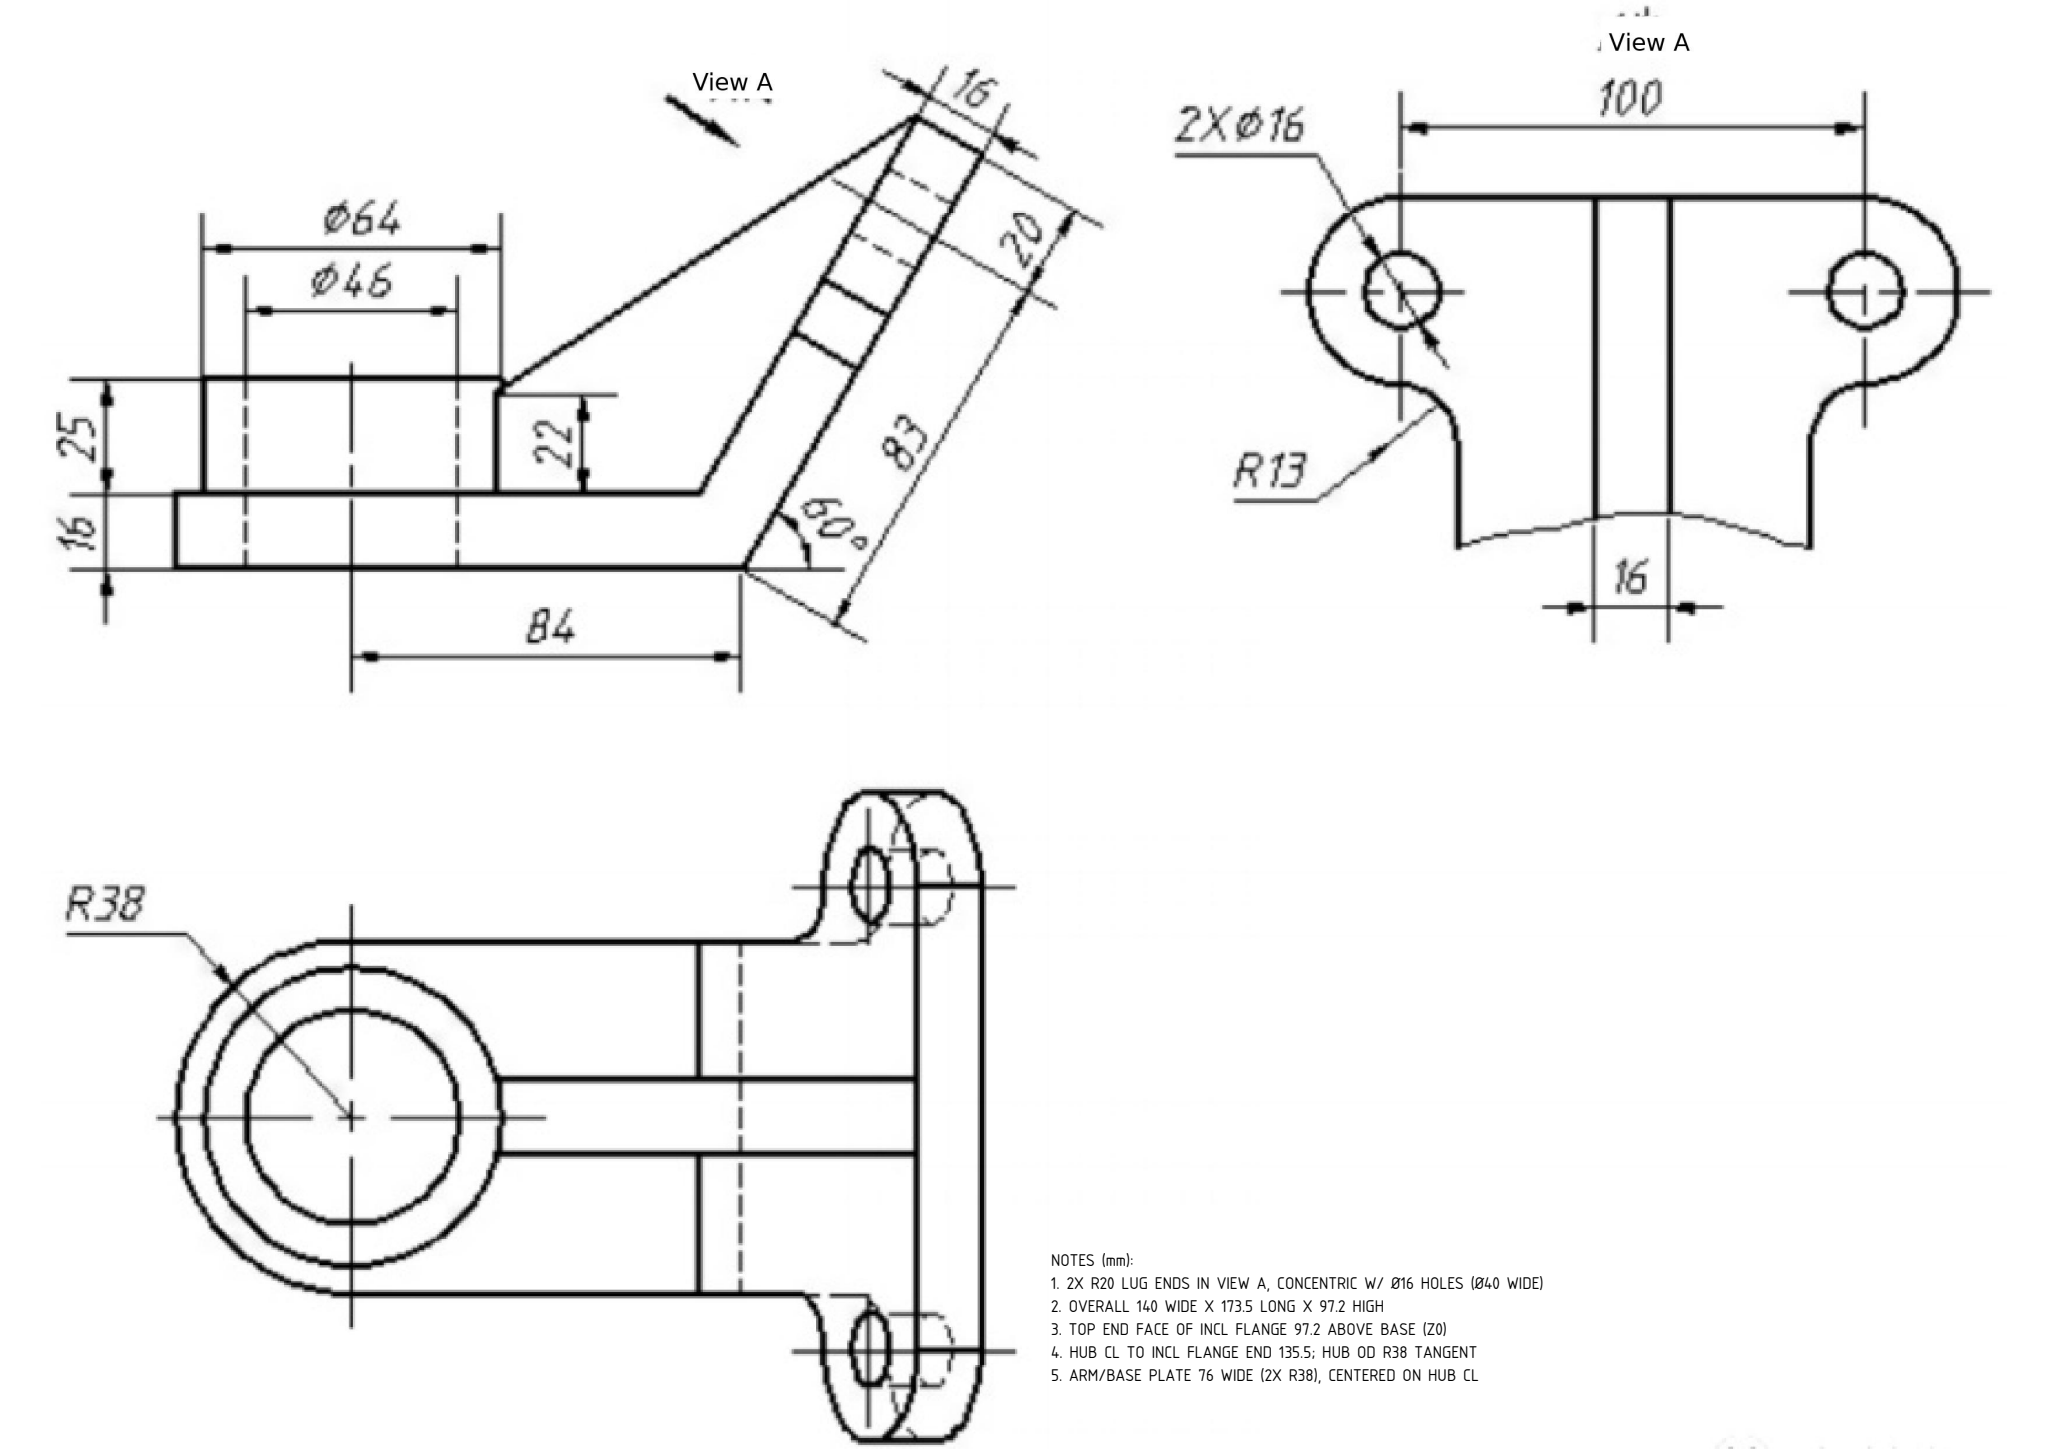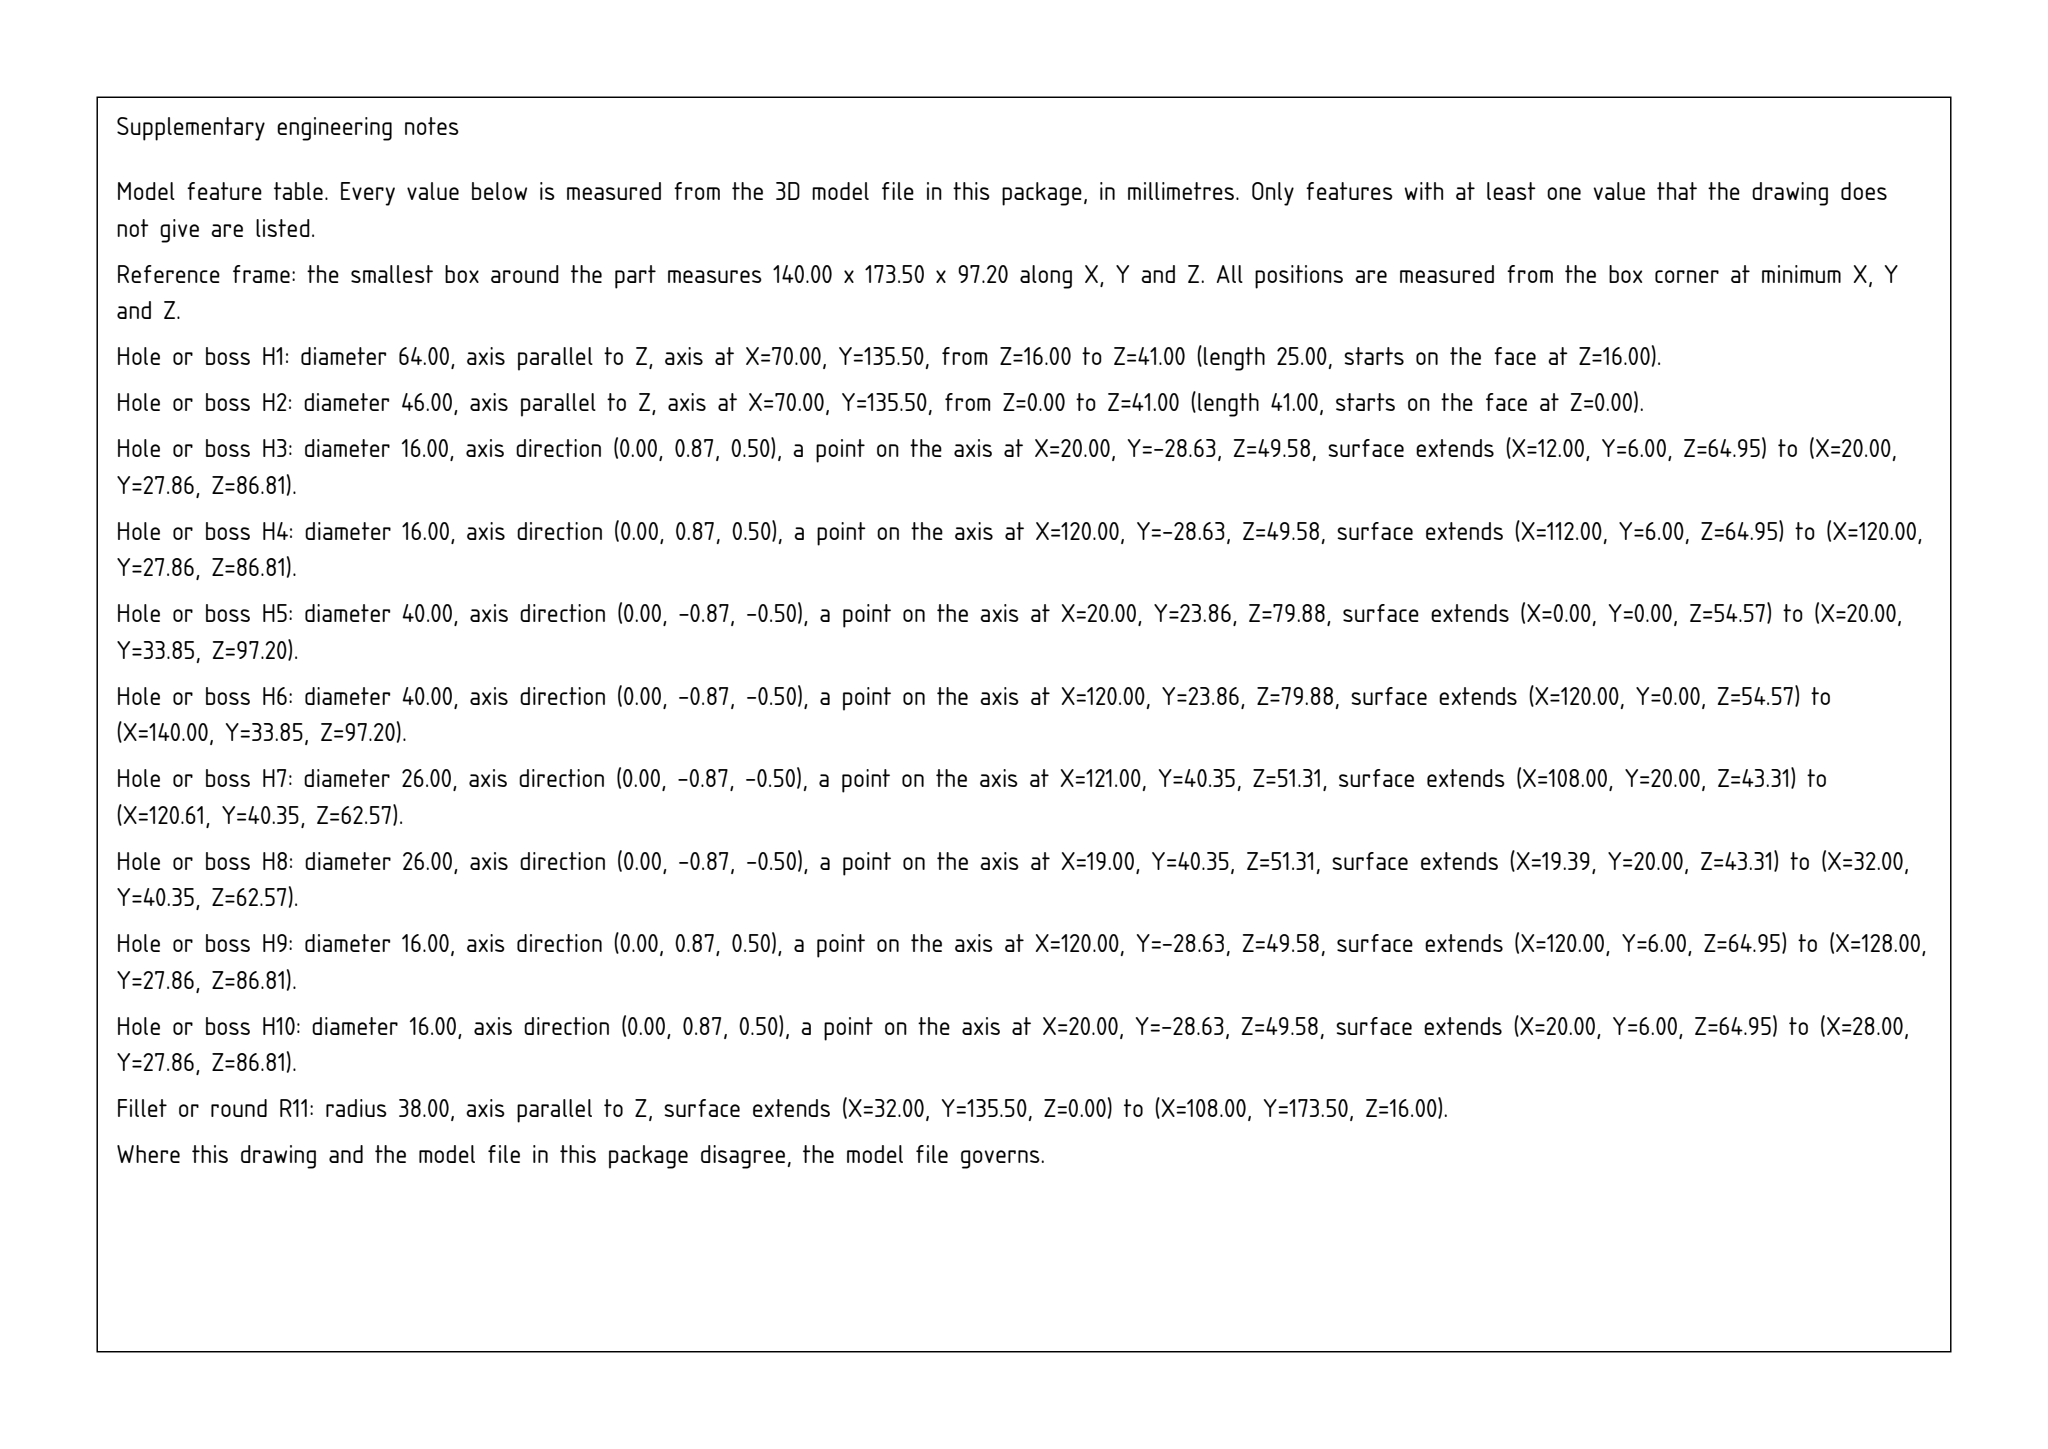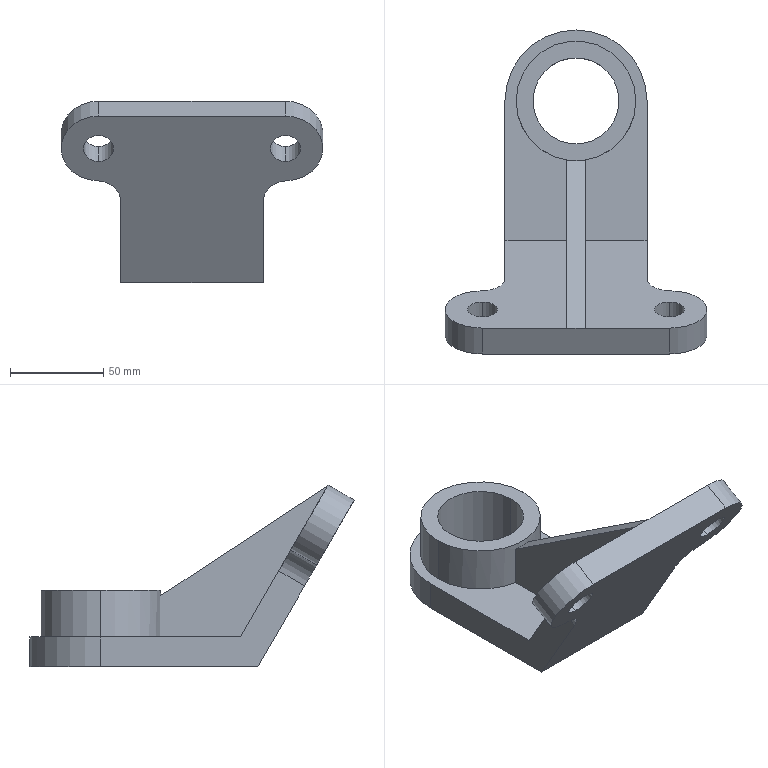Part | SolidWorks | mm | 1 solid | 25 faces | box 140 x 173.5 x 97.2 mm | volume 322175 mm3 | cylinder 13 | plane 12 | commonest cylinder face diameters 16 x4 46 x2 64 x2 40 x2 26 x2 76 x1
Drawing notes:
2X R20 LUG ENDS IN VIEW A, CONCENTRIC W/ Ø16 HOLES (Ø40 WIDE) | from the solid: Ø40 cyl, axis Y, at x=20 and x=120 (same x as the 2X Ø16 holes) -> R20 rounded lug ends, 100 apart
OVERALL 140 WIDE X 173.5 LONG X 97.2 HIGH | from the solid: bbox_xyz = [140.0, 173.5, 97.201]
TOP END FACE OF INCL FLANGE 97.2 ABOVE BASE (Z0) | from the solid: bbox Z max = 97.201 above base plane z=0; base bottom plane z=0.0
HUB CL TO INCL FLANGE END 135.5; HUB OD R38 TANGENT | from the solid: Ø46/Ø64/Ø76 hub axis at y=135.5 from bbox y-min; bbox y = 173.5 = 135.5 + 38
ARM/BASE PLATE 76 WIDE (2X R38), CENTERED ON HUB CL | from the solid: x-normal planes at 32.0 and 108.0 (76 apart) symmetric about hub axis x=70; Ø76 cyl, axis Z, pos (70,135.5), L=16
STEP:
#1=CARTESIAN_POINT('',(-50.,-121.5,64.952));
#2=VERTEX_POINT('',#1);
#3=CARTESIAN_POINT('',(-50.,-129.5,78.808));
#4=VERTEX_POINT('',#3);
#5=CARTESIAN_POINT('',(-50.,-125.5,71.88));
#6=DIRECTION('',(0.,0.866,0.5));
#7=DIRECTION('',(0.,-0.5,0.866));
#8=AXIS2_PLACEMENT_3D('',#5,#6,#7);
#9=CIRCLE('',#8,8.);
#10=EDGE_CURVE('',#2,#4,#9,.T.);
#11=ORIENTED_EDGE('',*,*,#10,.F.);
#12=CARTESIAN_POINT('',(-50.,-107.644,72.952));
#13=VERTEX_POINT('',#12);
#14=CARTESIAN_POINT('',(-50.,-160.125,42.652));
#15=DIRECTION('',(0.,0.866,0.5));
#16=VECTOR('',#15,1000.);
#17=LINE('',#14,#16);
#18=EDGE_CURVE('',#2,#13,#17,.T.);
#19=ORIENTED_EDGE('',*,*,#18,.T.);
#20=CARTESIAN_POINT('',(-50.,-115.644,86.808));
#21=VERTEX_POINT('',#20);
#22=CARTESIAN_POINT('',(-50.,-111.644,79.88));
#23=DIRECTION('',(0.,0.866,0.5));
#24=DIRECTION('',(0.,-0.5,0.866));
#25=AXIS2_PLACEMENT_3D('',#22,#23,#24);
#26=CIRCLE('',#25,8.);
#27=EDGE_CURVE('',#13,#21,#26,.T.);
#28=ORIENTED_EDGE('',*,*,#27,.T.);
#29=CARTESIAN_POINT('',(-50.,-168.125,56.508));
#30=DIRECTION('',(0.,0.866,0.5));
#31=VECTOR('',#30,1000.);
#32=LINE('',#29,#31);
#33=EDGE_CURVE('',#4,#21,#32,.T.);
#34=ORIENTED_EDGE('',*,*,#33,.F.);
#35=EDGE_LOOP('',(#11,#19,#28,#34));
#36=FACE_OUTER_BOUND('',#35,.T.);
#37=CARTESIAN_POINT('',(-50.,-164.125,49.58));
#38=DIRECTION('',(0.,0.866,0.5));
#39=DIRECTION('',(0.,-0.5,0.866));
#40=AXIS2_PLACEMENT_3D('',#37,#38,#39);
#41=CYLINDRICAL_SURFACE('',#40,8.);
#42=ADVANCED_FACE('',(#36),#41,.F.);
#43=CARTESIAN_POINT('',(50.,-121.5,64.952));
#44=VERTEX_POINT('',#43);
#45=CARTESIAN_POINT('',(50.,-129.5,78.808));
#46=VERTEX_POINT('',#45);
#47=CARTESIAN_POINT('',(50.,-125.5,71.88));
#48=DIRECTION('',(0.,0.866,0.5));
#49=DIRECTION('',(0.,-0.5,0.866));
#50=AXIS2_PLACEMENT_3D('',#47,#48,#49);
#51=CIRCLE('',#50,8.);
#52=EDGE_CURVE('',#44,#46,#51,.T.);
#53=ORIENTED_EDGE('',*,*,#52,.F.);
#54=CARTESIAN_POINT('',(50.,-107.644,72.952));
#55=VERTEX_POINT('',#54);
#56=CARTESIAN_POINT('',(50.,-160.125,42.652));
#57=DIRECTION('',(0.,0.866,0.5));
#58=VECTOR('',#57,1000.);
#59=LINE('',#56,#58);
#60=EDGE_CURVE('',#44,#55,#59,.T.);
#61=ORIENTED_EDGE('',*,*,#60,.T.);
#62=CARTESIAN_POINT('',(50.,-115.644,86.808));
#63=VERTEX_POINT('',#62);
#64=CARTESIAN_POINT('',(50.,-111.644,79.88));
#65=DIRECTION('',(0.,0.866,0.5));
#66=DIRECTION('',(0.,-0.5,0.866));
#67=AXIS2_PLACEMENT_3D('',#64,#65,#66);
#68=CIRCLE('',#67,8.);
#69=EDGE_CURVE('',#55,#63,#68,.T.);
#70=ORIENTED_EDGE('',*,*,#69,.T.);
#71=CARTESIAN_POINT('',(50.,-168.125,56.508));
#72=DIRECTION('',(0.,0.866,0.5));
#73=VECTOR('',#72,1000.);
#74=LINE('',#71,#73);
#75=EDGE_CURVE('',#46,#63,#74,.T.);
#76=ORIENTED_EDGE('',*,*,#75,.F.);
#77=EDGE_LOOP('',(#53,#61,#70,#76));
#78=FACE_OUTER_BOUND('',#77,.T.);
#79=CARTESIAN_POINT('',(50.,-164.125,49.58));
#80=DIRECTION('',(0.,0.866,0.5));
#81=DIRECTION('',(0.,-0.5,0.866));
#82=AXIS2_PLACEMENT_3D('',#79,#80,#81);
#83=CYLINDRICAL_SURFACE('',#82,8.);
#84=ADVANCED_FACE('',(#78),#83,.F.);
#85=CARTESIAN_POINT('',(-23.,0.,0.));
#86=VERTEX_POINT('',#85);
#87=CARTESIAN_POINT('',(23.,0.,0.));
#88=VERTEX_POINT('',#87);
#89=CARTESIAN_POINT('',(0.,0.,0.));
#90=DIRECTION('',(0.,0.,1.));
#91=DIRECTION('',(1.,0.,0.));
#92=AXIS2_PLACEMENT_3D('',#89,#90,#91);
#93=CIRCLE('',#92,23.);
#94=EDGE_CURVE('',#86,#88,#93,.T.);
#95=ORIENTED_EDGE('',*,*,#94,.F.);
#96=CARTESIAN_POINT('',(-23.,0.,41.));
#97=VERTEX_POINT('',#96);
#98=CARTESIAN_POINT('',(-23.,0.,0.));
#99=DIRECTION('',(0.,0.,1.));
#100=VECTOR('',#99,1000.);
#101=LINE('',#98,#100);
#102=EDGE_CURVE('',#86,#97,#101,.T.);
#103=ORIENTED_EDGE('',*,*,#102,.T.);
#104=CARTESIAN_POINT('',(23.,0.,41.));
#105=VERTEX_POINT('',#104);
#106=CARTESIAN_POINT('',(0.,0.,41.));
#107=DIRECTION('',(0.,0.,1.));
#108=DIRECTION('',(1.,0.,0.));
#109=AXIS2_PLACEMENT_3D('',#106,#107,#108);
#110=CIRCLE('',#109,23.);
#111=EDGE_CURVE('',#97,#105,#110,.T.);
#112=ORIENTED_EDGE('',*,*,#111,.T.);
#113=CARTESIAN_POINT('',(23.,0.,0.));
#114=DIRECTION('',(0.,0.,1.));
#115=VECTOR('',#114,1000.);
#116=LINE('',#113,#115);
#117=EDGE_CURVE('',#88,#105,#116,.T.);
#118=ORIENTED_EDGE('',*,*,#117,.F.);
#119=EDGE_LOOP('',(#95,#103,#112,#118));
#120=FACE_OUTER_BOUND('',#119,.T.);
#121=CARTESIAN_POINT('',(0.,0.,0.));
#122=DIRECTION('',(0.,0.,1.));
#123=DIRECTION('',(1.,0.,0.));
#124=AXIS2_PLACEMENT_3D('',#121,#122,#123);
#125=CYLINDRICAL_SURFACE('',#124,23.);
#126=ADVANCED_FACE('',(#120),#125,.F.);
#127=CARTESIAN_POINT('',(32.,0.,41.));
#128=VERTEX_POINT('',#127);
#129=CARTESIAN_POINT('',(-32.,0.,41.));
#130=VERTEX_POINT('',#129);
#131=CARTESIAN_POINT('',(0.,0.,41.));
#132=DIRECTION('',(0.,0.,1.));
#133=DIRECTION('',(1.,0.,0.));
#134=AXIS2_PLACEMENT_3D('',#131,#132,#133);
#135=CIRCLE('',#134,32.);
#136=EDGE_CURVE('',#128,#130,#135,.T.);
#137=ORIENTED_EDGE('',*,*,#136,.F.);
#138=CARTESIAN_POINT('',(32.,0.,16.));
#139=VERTEX_POINT('',#138);
#140=CARTESIAN_POINT('',(32.,0.,41.));
#141=DIRECTION('',(0.,0.,-1.));
#142=VECTOR('',#141,1000.);
#143=LINE('',#140,#142);
#144=EDGE_CURVE('',#128,#139,#143,.T.);
#145=ORIENTED_EDGE('',*,*,#144,.T.);
#146=CARTESIAN_POINT('',(-32.,0.,16.));
#147=VERTEX_POINT('',#146);
#148=CARTESIAN_POINT('',(0.,0.,16.));
#149=DIRECTION('',(0.,0.,1.));
#150=DIRECTION('',(1.,0.,0.));
#151=AXIS2_PLACEMENT_3D('',#148,#149,#150);
#152=CIRCLE('',#151,32.);
#153=EDGE_CURVE('',#139,#147,#152,.T.);
#154=ORIENTED_EDGE('',*,*,#153,.T.);
#155=CARTESIAN_POINT('',(-32.,0.,41.));
#156=DIRECTION('',(0.,0.,-1.));
#157=VECTOR('',#156,1000.);
#158=LINE('',#155,#157);
#159=EDGE_CURVE('',#130,#147,#158,.T.);
#160=ORIENTED_EDGE('',*,*,#159,.F.);
#161=EDGE_LOOP('',(#137,#145,#154,#160));
#162=FACE_OUTER_BOUND('',#161,.T.);
#163=CARTESIAN_POINT('',(0.,0.,41.));
#164=DIRECTION('',(0.,0.,-1.));
#165=DIRECTION('',(-1.,0.,0.));
#166=AXIS2_PLACEMENT_3D('',#163,#164,#165);
#167=CYLINDRICAL_SURFACE('',#166,32.);
#168=ADVANCED_FACE('',(#162),#167,.T.);
#169=CARTESIAN_POINT('',(-50.,-111.644,79.88));
#170=DIRECTION('',(0.,0.866,0.5));
#171=DIRECTION('',(0.,-0.5,0.866));
#172=AXIS2_PLACEMENT_3D('',#169,#170,#171);
#173=CIRCLE('',#172,8.);
#174=EDGE_CURVE('',#21,#13,#173,.T.);
#175=ORIENTED_EDGE('',*,*,#174,.F.);
#176=ORIENTED_EDGE('',*,*,#27,.F.);
#177=EDGE_LOOP('',(#175,#176));
#178=FACE_BOUND('',#177,.T.);
#179=CARTESIAN_POINT('',(-50.,-121.644,97.201));
#180=VERTEX_POINT('',#179);
#181=CARTESIAN_POINT('',(-5.,-121.644,97.201));
#182=VERTEX_POINT('',#181);
#183=CARTESIAN_POINT('',(-50.,-121.644,97.201));
#184=DIRECTION('',(1.,0.,0.));
#185=VECTOR('',#184,1000.);
#186=LINE('',#183,#185);
#187=EDGE_CURVE('',#180,#182,#186,.T.);
#188=ORIENTED_EDGE('',*,*,#187,.T.);
#189=CARTESIAN_POINT('',(-5.,-74.762,16.));
#190=VERTEX_POINT('',#189);
#191=CARTESIAN_POINT('',(-5.,-111.644,79.88));
#192=DIRECTION('',(0.,0.5,-0.866));
#193=VECTOR('',#192,1000.);
#194=LINE('',#191,#193);
#195=EDGE_CURVE('',#182,#190,#194,.T.);
#196=ORIENTED_EDGE('',*,*,#195,.T.);
#197=CARTESIAN_POINT('',(-38.,-74.762,16.));
#198=VERTEX_POINT('',#197);
#199=CARTESIAN_POINT('',(0.,-74.762,16.));
#200=DIRECTION('',(-1.,0.,0.));
#201=VECTOR('',#200,1000.);
#202=LINE('',#199,#201);
#203=EDGE_CURVE('',#190,#198,#202,.T.);
#204=ORIENTED_EDGE('',*,*,#203,.T.);
#205=CARTESIAN_POINT('',(-38.,-95.151,51.314));
#206=VERTEX_POINT('',#205);
#207=CARTESIAN_POINT('',(-38.,-70.144,8.));
#208=DIRECTION('',(0.,-0.5,0.866));
#209=VECTOR('',#208,1000.);
#210=LINE('',#207,#209);
#211=EDGE_CURVE('',#198,#206,#210,.T.);
#212=ORIENTED_EDGE('',*,*,#211,.T.);
#213=CARTESIAN_POINT('',(-50.606,-101.648,62.568));
#214=VERTEX_POINT('',#213);
#215=CARTESIAN_POINT('',(-51.,-95.151,51.314));
#216=DIRECTION('',(0.,0.866,0.5));
#217=DIRECTION('',(0.,-0.5,0.866));
#218=AXIS2_PLACEMENT_3D('',#215,#216,#217);
#219=CIRCLE('',#218,13.);
#220=EDGE_CURVE('',#214,#206,#219,.T.);
#221=ORIENTED_EDGE('',*,*,#220,.F.);
#222=CARTESIAN_POINT('',(-50.,-111.644,79.88));
#223=DIRECTION('',(0.,0.866,0.5));
#224=DIRECTION('',(0.,-0.5,0.866));
#225=AXIS2_PLACEMENT_3D('',#222,#223,#224);
#226=CIRCLE('',#225,20.);
#227=EDGE_CURVE('',#214,#180,#226,.T.);
#228=ORIENTED_EDGE('',*,*,#227,.T.);
#229=EDGE_LOOP('',(#188,#196,#204,#212,#221,#228));
#230=FACE_OUTER_BOUND('',#229,.T.);
#231=CARTESIAN_POINT('',(-50.,-111.644,79.88));
#232=DIRECTION('',(0.,0.866,0.5));
#233=DIRECTION('',(0.,-0.5,0.866));
#234=AXIS2_PLACEMENT_3D('',#231,#232,#233);
#235=PLANE('',#234);
#236=ADVANCED_FACE('',(#178,#230),#235,.T.);
#237=CARTESIAN_POINT('',(38.,0.,0.));
#238=VERTEX_POINT('',#237);
#239=CARTESIAN_POINT('',(-38.,0.,0.));
#240=VERTEX_POINT('',#239);
#241=CARTESIAN_POINT('',(0.,0.,0.));
#242=DIRECTION('',(0.,0.,1.));
#243=DIRECTION('',(1.,0.,0.));
#244=AXIS2_PLACEMENT_3D('',#241,#242,#243);
#245=CIRCLE('',#244,38.);
#246=EDGE_CURVE('',#238,#240,#245,.T.);
#247=ORIENTED_EDGE('',*,*,#246,.T.);
#248=CARTESIAN_POINT('',(-38.,0.,16.));
#249=VERTEX_POINT('',#248);
#250=CARTESIAN_POINT('',(-38.,0.,16.));
#251=DIRECTION('',(0.,0.,-1.));
#252=VECTOR('',#251,1000.);
#253=LINE('',#250,#252);
#254=EDGE_CURVE('',#249,#240,#253,.T.);
#255=ORIENTED_EDGE('',*,*,#254,.F.);
#256=CARTESIAN_POINT('',(38.,0.,16.));
#257=VERTEX_POINT('',#256);
#258=CARTESIAN_POINT('',(0.,0.,16.));
#259=DIRECTION('',(0.,0.,1.));
#260=DIRECTION('',(1.,0.,0.));
#261=AXIS2_PLACEMENT_3D('',#258,#259,#260);
#262=CIRCLE('',#261,38.);
#263=EDGE_CURVE('',#257,#249,#262,.T.);
#264=ORIENTED_EDGE('',*,*,#263,.F.);
#265=CARTESIAN_POINT('',(38.,0.,16.));
#266=DIRECTION('',(0.,0.,-1.));
#267=VECTOR('',#266,1000.);
#268=LINE('',#265,#267);
#269=EDGE_CURVE('',#257,#238,#268,.T.);
#270=ORIENTED_EDGE('',*,*,#269,.T.);
#271=EDGE_LOOP('',(#247,#255,#264,#270));
#272=FACE_OUTER_BOUND('',#271,.T.);
#273=CARTESIAN_POINT('',(0.,0.,16.));
#274=DIRECTION('',(0.,0.,-1.));
#275=DIRECTION('',(-1.,0.,0.));
#276=AXIS2_PLACEMENT_3D('',#273,#274,#275);
#277=CYLINDRICAL_SURFACE('',#276,38.);
#278=ADVANCED_FACE('',(#272),#277,.T.);
#279=CARTESIAN_POINT('',(-38.,-84.,0.));
#280=VERTEX_POINT('',#279);
#281=CARTESIAN_POINT('',(-38.,-84.,0.));
#282=DIRECTION('',(-0.,-1.,0.));
#283=VECTOR('',#282,1000.);
#284=LINE('',#281,#283);
#285=EDGE_CURVE('',#240,#280,#284,.T.);
#286=ORIENTED_EDGE('',*,*,#285,.T.);
#287=CARTESIAN_POINT('',(-38.,-109.008,43.314));
#288=VERTEX_POINT('',#287);
#289=CARTESIAN_POINT('',(-38.,-84.,0.));
#290=DIRECTION('',(0.,-0.5,0.866));
#291=VECTOR('',#290,1000.);
#292=LINE('',#289,#291);
#293=EDGE_CURVE('',#280,#288,#292,.T.);
#294=ORIENTED_EDGE('',*,*,#293,.T.);
#295=CARTESIAN_POINT('',(-38.,-95.151,51.314));
#296=DIRECTION('',(0.,-0.866,-0.5));
#297=VECTOR('',#296,1000.);
#298=LINE('',#295,#297);
#299=EDGE_CURVE('',#206,#288,#298,.T.);
#300=ORIENTED_EDGE('',*,*,#299,.F.);
#301=ORIENTED_EDGE('',*,*,#211,.F.);
#302=CARTESIAN_POINT('',(-38.,-84.,16.));
#303=DIRECTION('',(-0.,-1.,0.));
#304=VECTOR('',#303,1000.);
#305=LINE('',#302,#304);
#306=EDGE_CURVE('',#249,#198,#305,.T.);
#307=ORIENTED_EDGE('',*,*,#306,.F.);
#308=ORIENTED_EDGE('',*,*,#254,.T.);
#309=EDGE_LOOP('',(#286,#294,#300,#301,#307,#308));
#310=FACE_OUTER_BOUND('',#309,.T.);
#311=CARTESIAN_POINT('',(-38.,-84.,16.));
#312=DIRECTION('',(1.,-0.,0.));
#313=DIRECTION('',(0.,1.,0.));
#314=AXIS2_PLACEMENT_3D('',#311,#312,#313);
#315=PLANE('',#314);
#316=ADVANCED_FACE('',(#310),#315,.F.);
#317=CARTESIAN_POINT('',(38.,-84.,0.));
#318=VERTEX_POINT('',#317);
#319=CARTESIAN_POINT('',(38.,-109.008,43.314));
#320=VERTEX_POINT('',#319);
#321=CARTESIAN_POINT('',(38.,-84.,0.));
#322=DIRECTION('',(-0.,-0.5,0.866));
#323=VECTOR('',#322,1000.);
#324=LINE('',#321,#323);
#325=EDGE_CURVE('',#318,#320,#324,.T.);
#326=ORIENTED_EDGE('',*,*,#325,.F.);
#327=CARTESIAN_POINT('',(38.,0.,0.));
#328=DIRECTION('',(-0.,1.,0.));
#329=VECTOR('',#328,1000.);
#330=LINE('',#327,#329);
#331=EDGE_CURVE('',#318,#238,#330,.T.);
#332=ORIENTED_EDGE('',*,*,#331,.T.);
#333=ORIENTED_EDGE('',*,*,#269,.F.);
#334=CARTESIAN_POINT('',(38.,-74.762,16.));
#335=VERTEX_POINT('',#334);
#336=CARTESIAN_POINT('',(38.,0.,16.));
#337=DIRECTION('',(-0.,1.,0.));
#338=VECTOR('',#337,1000.);
#339=LINE('',#336,#338);
#340=EDGE_CURVE('',#335,#257,#339,.T.);
#341=ORIENTED_EDGE('',*,*,#340,.F.);
#342=CARTESIAN_POINT('',(38.,-95.151,51.314));
#343=VERTEX_POINT('',#342);
#344=CARTESIAN_POINT('',(38.,-70.144,8.));
#345=DIRECTION('',(-0.,-0.5,0.866));
#346=VECTOR('',#345,1000.);
#347=LINE('',#344,#346);
#348=EDGE_CURVE('',#335,#343,#347,.T.);
#349=ORIENTED_EDGE('',*,*,#348,.T.);
#350=CARTESIAN_POINT('',(38.,-95.151,51.314));
#351=DIRECTION('',(0.,-0.866,-0.5));
#352=VECTOR('',#351,1000.);
#353=LINE('',#350,#352);
#354=EDGE_CURVE('',#343,#320,#353,.T.);
#355=ORIENTED_EDGE('',*,*,#354,.T.);
#356=EDGE_LOOP('',(#326,#332,#333,#341,#349,#355));
#357=FACE_OUTER_BOUND('',#356,.T.);
#358=CARTESIAN_POINT('',(38.,0.,16.));
#359=DIRECTION('',(-1.,-0.,0.));
#360=DIRECTION('',(0.,-1.,0.));
#361=AXIS2_PLACEMENT_3D('',#358,#359,#360);
#362=PLANE('',#361);
#363=ADVANCED_FACE('',(#357),#362,.F.);
#364=CARTESIAN_POINT('',(5.,-74.762,16.));
#365=VERTEX_POINT('',#364);
#366=CARTESIAN_POINT('',(5.,-31.607,16.));
#367=VERTEX_POINT('',#366);
#368=CARTESIAN_POINT('',(5.,0.,16.));
#369=DIRECTION('',(0.,1.,0.));
#370=VECTOR('',#369,1000.);
#371=LINE('',#368,#370);
#372=EDGE_CURVE('',#365,#367,#371,.T.);
#373=ORIENTED_EDGE('',*,*,#372,.F.);
#374=CARTESIAN_POINT('',(0.,-74.762,16.));
#375=DIRECTION('',(-1.,0.,0.));
#376=VECTOR('',#375,1000.);
#377=LINE('',#374,#376);
#378=EDGE_CURVE('',#335,#365,#377,.T.);
#379=ORIENTED_EDGE('',*,*,#378,.F.);
#380=ORIENTED_EDGE('',*,*,#340,.T.);
#381=ORIENTED_EDGE('',*,*,#263,.T.);
#382=ORIENTED_EDGE('',*,*,#306,.T.);
#383=ORIENTED_EDGE('',*,*,#203,.F.);
#384=CARTESIAN_POINT('',(-5.,-31.607,16.));
#385=VERTEX_POINT('',#384);
#386=CARTESIAN_POINT('',(-5.,0.,16.));
#387=DIRECTION('',(0.,1.,0.));
#388=VECTOR('',#387,1000.);
#389=LINE('',#386,#388);
#390=EDGE_CURVE('',#190,#385,#389,.T.);
#391=ORIENTED_EDGE('',*,*,#390,.T.);
#392=CARTESIAN_POINT('',(0.,0.,16.));
#393=DIRECTION('',(0.,0.,1.));
#394=DIRECTION('',(1.,0.,0.));
#395=AXIS2_PLACEMENT_3D('',#392,#393,#394);
#396=CIRCLE('',#395,32.);
#397=EDGE_CURVE('',#147,#385,#396,.T.);
#398=ORIENTED_EDGE('',*,*,#397,.F.);
#399=ORIENTED_EDGE('',*,*,#153,.F.);
#400=CARTESIAN_POINT('',(0.,0.,16.));
#401=DIRECTION('',(0.,0.,1.));
#402=DIRECTION('',(1.,0.,0.));
#403=AXIS2_PLACEMENT_3D('',#400,#401,#402);
#404=CIRCLE('',#403,32.);
#405=EDGE_CURVE('',#367,#139,#404,.T.);
#406=ORIENTED_EDGE('',*,*,#405,.F.);
#407=EDGE_LOOP('',(#373,#379,#380,#381,#382,#383,#391,#398,#399,#406));
#408=FACE_OUTER_BOUND('',#407,.T.);
#409=CARTESIAN_POINT('',(0.,0.,16.));
#410=DIRECTION('',(0.,0.,1.));
#411=DIRECTION('',(1.,0.,0.));
#412=AXIS2_PLACEMENT_3D('',#409,#410,#411);
#413=PLANE('',#412);
#414=ADVANCED_FACE('',(#408),#413,.T.);
#415=CARTESIAN_POINT('',(0.,0.,0.));
#416=DIRECTION('',(0.,0.,1.));
#417=DIRECTION('',(1.,0.,0.));
#418=AXIS2_PLACEMENT_3D('',#415,#416,#417);
#419=CIRCLE('',#418,23.);
#420=EDGE_CURVE('',#88,#86,#419,.T.);
#421=ORIENTED_EDGE('',*,*,#420,.T.);
#422=ORIENTED_EDGE('',*,*,#94,.T.);
#423=EDGE_LOOP('',(#421,#422));
#424=FACE_BOUND('',#423,.T.);
#425=ORIENTED_EDGE('',*,*,#331,.F.);
#426=CARTESIAN_POINT('',(38.,-84.,0.));
#427=DIRECTION('',(1.,0.,0.));
#428=VECTOR('',#427,1000.);
#429=LINE('',#426,#428);
#430=EDGE_CURVE('',#280,#318,#429,.T.);
#431=ORIENTED_EDGE('',*,*,#430,.F.);
#432=ORIENTED_EDGE('',*,*,#285,.F.);
#433=ORIENTED_EDGE('',*,*,#246,.F.);
#434=EDGE_LOOP('',(#425,#431,#432,#433));
#435=FACE_OUTER_BOUND('',#434,.T.);
#436=CARTESIAN_POINT('',(0.,0.,0.));
#437=DIRECTION('',(0.,0.,1.));
#438=DIRECTION('',(1.,0.,0.));
#439=AXIS2_PLACEMENT_3D('',#436,#437,#438);
#440=PLANE('',#439);
#441=ADVANCED_FACE('',(#424,#435),#440,.F.);
#442=ORIENTED_EDGE('',*,*,#144,.F.);
#443=CARTESIAN_POINT('',(0.,0.,41.));
#444=DIRECTION('',(0.,0.,1.));
#445=DIRECTION('',(1.,0.,0.));
#446=AXIS2_PLACEMENT_3D('',#443,#444,#445);
#447=CIRCLE('',#446,32.);
#448=EDGE_CURVE('',#130,#128,#447,.T.);
#449=ORIENTED_EDGE('',*,*,#448,.F.);
#450=ORIENTED_EDGE('',*,*,#159,.T.);
#451=ORIENTED_EDGE('',*,*,#397,.T.);
#452=CARTESIAN_POINT('',(-5.,-31.607,37.74));
#453=VERTEX_POINT('',#452);
#454=CARTESIAN_POINT('',(-5.,-31.607,41.));
#455=DIRECTION('',(0.,0.,-1.));
#456=VECTOR('',#455,1000.);
#457=LINE('',#454,#456);
#458=EDGE_CURVE('',#453,#385,#457,.T.);
#459=ORIENTED_EDGE('',*,*,#458,.F.);
#460=CARTESIAN_POINT('',(5.,-31.607,37.74));
#461=VERTEX_POINT('',#460);
#462=CARTESIAN_POINT('',(-5.,-31.607,37.74));
#463=CARTESIAN_POINT('',(-1.68,-32.132,38.087));
#464=CARTESIAN_POINT('',(1.68,-32.132,38.087));
#465=CARTESIAN_POINT('',(5.,-31.607,37.74));
#466=(BOUNDED_CURVE()B_SPLINE_CURVE(3,(#462,#463,#464,#465),.UNSPECIFIED.,.F.,.F.)B_SPLINE_CURVE_WITH_KNOTS((4,4),(2.985,3.298),.UNSPECIFIED.)CURVE()GEOMETRIC_REPRESENTATION_ITEM()RATIONAL_B_SPLINE_CURVE((1.,0.9918,0.9918,1.))REPRESENTATION_ITEM(''));
#467=EDGE_CURVE('',#453,#461,#466,.T.);
#468=ORIENTED_EDGE('',*,*,#467,.T.);
#469=CARTESIAN_POINT('',(5.,-31.607,41.));
#470=DIRECTION('',(0.,0.,-1.));
#471=VECTOR('',#470,1000.);
#472=LINE('',#469,#471);
#473=EDGE_CURVE('',#461,#367,#472,.T.);
#474=ORIENTED_EDGE('',*,*,#473,.T.);
#475=ORIENTED_EDGE('',*,*,#405,.T.);
#476=EDGE_LOOP('',(#442,#449,#450,#451,#459,#468,#474,#475));
#477=FACE_OUTER_BOUND('',#476,.T.);
#478=CARTESIAN_POINT('',(0.,0.,41.));
#479=DIRECTION('',(0.,0.,-1.));
#480=DIRECTION('',(-1.,0.,0.));
#481=AXIS2_PLACEMENT_3D('',#478,#479,#480);
#482=CYLINDRICAL_SURFACE('',#481,32.);
#483=ADVANCED_FACE('',(#477),#482,.T.);
#484=CARTESIAN_POINT('',(0.,0.,41.));
#485=DIRECTION('',(0.,0.,1.));
#486=DIRECTION('',(1.,0.,0.));
#487=AXIS2_PLACEMENT_3D('',#484,#485,#486);
#488=CIRCLE('',#487,23.);
#489=EDGE_CURVE('',#105,#97,#488,.T.);
#490=ORIENTED_EDGE('',*,*,#489,.F.);
#491=ORIENTED_EDGE('',*,*,#111,.F.);
#492=EDGE_LOOP('',(#490,#491));
#493=FACE_BOUND('',#492,.T.);
#494=ORIENTED_EDGE('',*,*,#448,.T.);
#495=ORIENTED_EDGE('',*,*,#136,.T.);
#496=EDGE_LOOP('',(#494,#495));
#497=FACE_OUTER_BOUND('',#496,.T.);
#498=CARTESIAN_POINT('',(0.,0.,41.));
#499=DIRECTION('',(0.,0.,1.));
#500=DIRECTION('',(1.,0.,0.));
#501=AXIS2_PLACEMENT_3D('',#498,#499,#500);
#502=PLANE('',#501);
#503=ADVANCED_FACE('',(#493,#497),#502,.T.);
#504=CARTESIAN_POINT('',(-50.606,-115.505,54.568));
#505=VERTEX_POINT('',#504);
#506=CARTESIAN_POINT('',(-50.,-135.5,89.201));
#507=VERTEX_POINT('',#506);
#508=CARTESIAN_POINT('',(-50.,-125.5,71.88));
#509=DIRECTION('',(0.,0.866,0.5));
#510=DIRECTION('',(0.,-0.5,0.866));
#511=AXIS2_PLACEMENT_3D('',#508,#509,#510);
#512=CIRCLE('',#511,20.);
#513=EDGE_CURVE('',#505,#507,#512,.T.);
#514=ORIENTED_EDGE('',*,*,#513,.T.);
#515=CARTESIAN_POINT('',(-50.,-121.644,97.201));
#516=DIRECTION('',(0.,-0.866,-0.5));
#517=VECTOR('',#516,1000.);
#518=LINE('',#515,#517);
#519=EDGE_CURVE('',#180,#507,#518,.T.);
#520=ORIENTED_EDGE('',*,*,#519,.F.);
#521=ORIENTED_EDGE('',*,*,#227,.F.);
#522=CARTESIAN_POINT('',(-50.606,-101.648,62.568));
#523=DIRECTION('',(0.,-0.866,-0.5));
#524=VECTOR('',#523,1000.);
#525=LINE('',#522,#524);
#526=EDGE_CURVE('',#214,#505,#525,.T.);
#527=ORIENTED_EDGE('',*,*,#526,.T.);
#528=EDGE_LOOP('',(#514,#520,#521,#527));
#529=FACE_OUTER_BOUND('',#528,.T.);
#530=CARTESIAN_POINT('',(-50.,-111.644,79.88));
#531=DIRECTION('',(0.,-0.866,-0.5));
#532=DIRECTION('',(0.,0.5,-0.866));
#533=AXIS2_PLACEMENT_3D('',#530,#531,#532);
#534=CYLINDRICAL_SURFACE('',#533,20.);
#535=ADVANCED_FACE('',(#529),#534,.T.);
#536=CARTESIAN_POINT('',(5.,-121.644,97.201));
#537=VERTEX_POINT('',#536);
#538=CARTESIAN_POINT('',(50.,-121.644,97.201));
#539=VERTEX_POINT('',#538);
#540=CARTESIAN_POINT('',(-50.,-121.644,97.201));
#541=DIRECTION('',(1.,0.,0.));
#542=VECTOR('',#541,1000.);
#543=LINE('',#540,#542);
#544=EDGE_CURVE('',#537,#539,#543,.T.);
#545=ORIENTED_EDGE('',*,*,#544,.F.);
#546=CARTESIAN_POINT('',(-50.,-121.644,97.201));
#547=DIRECTION('',(1.,0.,0.));
#548=VECTOR('',#547,1000.);
#549=LINE('',#546,#548);
#550=EDGE_CURVE('',#182,#537,#549,.T.);
#551=ORIENTED_EDGE('',*,*,#550,.F.);
#552=ORIENTED_EDGE('',*,*,#187,.F.);
#553=ORIENTED_EDGE('',*,*,#519,.T.);
#554=CARTESIAN_POINT('',(50.,-135.5,89.201));
#555=VERTEX_POINT('',#554);
#556=CARTESIAN_POINT('',(-50.,-135.5,89.201));
#557=DIRECTION('',(1.,0.,0.));
#558=VECTOR('',#557,1000.);
#559=LINE('',#556,#558);
#560=EDGE_CURVE('',#507,#555,#559,.T.);
#561=ORIENTED_EDGE('',*,*,#560,.T.);
#562=CARTESIAN_POINT('',(50.,-121.644,97.201));
#563=DIRECTION('',(0.,-0.866,-0.5));
#564=VECTOR('',#563,1000.);
#565=LINE('',#562,#564);
#566=EDGE_CURVE('',#539,#555,#565,.T.);
#567=ORIENTED_EDGE('',*,*,#566,.F.);
#568=EDGE_LOOP('',(#545,#551,#552,#553,#561,#567));
#569=FACE_OUTER_BOUND('',#568,.T.);
#570=CARTESIAN_POINT('',(-50.,-121.644,97.201));
#571=DIRECTION('',(0.,0.5,-0.866));
#572=DIRECTION('',(0.,0.866,0.5));
#573=AXIS2_PLACEMENT_3D('',#570,#571,#572);
#574=PLANE('',#573);
#575=ADVANCED_FACE('',(#569),#574,.F.);
#576=CARTESIAN_POINT('',(50.606,-115.505,54.568));
#577=VERTEX_POINT('',#576);
#578=CARTESIAN_POINT('',(50.,-125.5,71.88));
#579=DIRECTION('',(0.,-0.866,-0.5));
#580=DIRECTION('',(0.,0.5,-0.866));
#581=AXIS2_PLACEMENT_3D('',#578,#579,#580);
#582=CIRCLE('',#581,20.);
#583=EDGE_CURVE('',#577,#555,#582,.T.);
#584=ORIENTED_EDGE('',*,*,#583,.F.);
#585=CARTESIAN_POINT('',(50.606,-101.648,62.568));
#586=VERTEX_POINT('',#585);
#587=CARTESIAN_POINT('',(50.606,-101.648,62.568));
#588=DIRECTION('',(0.,-0.866,-0.5));
#589=VECTOR('',#588,1000.);
#590=LINE('',#587,#589);
#591=EDGE_CURVE('',#586,#577,#590,.T.);
#592=ORIENTED_EDGE('',*,*,#591,.F.);
#593=CARTESIAN_POINT('',(50.,-111.644,79.88));
#594=DIRECTION('',(0.,-0.866,-0.5));
#595=DIRECTION('',(0.,0.5,-0.866));
#596=AXIS2_PLACEMENT_3D('',#593,#594,#595);
#597=CIRCLE('',#596,20.);
#598=EDGE_CURVE('',#586,#539,#597,.T.);
#599=ORIENTED_EDGE('',*,*,#598,.T.);
#600=ORIENTED_EDGE('',*,*,#566,.T.);
#601=EDGE_LOOP('',(#584,#592,#599,#600));
#602=FACE_OUTER_BOUND('',#601,.T.);
#603=CARTESIAN_POINT('',(50.,-111.644,79.88));
#604=DIRECTION('',(0.,-0.866,-0.5));
#605=DIRECTION('',(0.,0.5,-0.866));
#606=AXIS2_PLACEMENT_3D('',#603,#604,#605);
#607=CYLINDRICAL_SURFACE('',#606,20.);
#608=ADVANCED_FACE('',(#602),#607,.T.);
#609=CARTESIAN_POINT('',(51.,-109.008,43.314));
#610=DIRECTION('',(0.,-0.866,-0.5));
#611=DIRECTION('',(0.,0.5,-0.866));
#612=AXIS2_PLACEMENT_3D('',#609,#610,#611);
#613=CIRCLE('',#612,13.);
#614=EDGE_CURVE('',#577,#320,#613,.T.);
#615=ORIENTED_EDGE('',*,*,#614,.T.);
#616=ORIENTED_EDGE('',*,*,#354,.F.);
#617=CARTESIAN_POINT('',(51.,-95.151,51.314));
#618=DIRECTION('',(0.,-0.866,-0.5));
#619=DIRECTION('',(0.,0.5,-0.866));
#620=AXIS2_PLACEMENT_3D('',#617,#618,#619);
#621=CIRCLE('',#620,13.);
#622=EDGE_CURVE('',#586,#343,#621,.T.);
#623=ORIENTED_EDGE('',*,*,#622,.F.);
#624=ORIENTED_EDGE('',*,*,#591,.T.);
#625=EDGE_LOOP('',(#615,#616,#623,#624));
#626=FACE_OUTER_BOUND('',#625,.T.);
#627=CARTESIAN_POINT('',(51.,-95.151,51.314));
#628=DIRECTION('',(0.,-0.866,-0.5));
#629=DIRECTION('',(0.,0.5,-0.866));
#630=AXIS2_PLACEMENT_3D('',#627,#628,#629);
#631=CYLINDRICAL_SURFACE('',#630,13.);
#632=ADVANCED_FACE('',(#626),#631,.F.);
#633=CARTESIAN_POINT('',(-51.,-109.008,43.314));
#634=DIRECTION('',(0.,0.866,0.5));
#635=DIRECTION('',(0.,-0.5,0.866));
#636=AXIS2_PLACEMENT_3D('',#633,#634,#635);
#637=CIRCLE('',#636,13.);
#638=EDGE_CURVE('',#505,#288,#637,.T.);
#639=ORIENTED_EDGE('',*,*,#638,.F.);
#640=ORIENTED_EDGE('',*,*,#526,.F.);
#641=ORIENTED_EDGE('',*,*,#220,.T.);
#642=ORIENTED_EDGE('',*,*,#299,.T.);
#643=EDGE_LOOP('',(#639,#640,#641,#642));
#644=FACE_OUTER_BOUND('',#643,.T.);
#645=CARTESIAN_POINT('',(-51.,-95.151,51.314));
#646=DIRECTION('',(0.,-0.866,-0.5));
#647=DIRECTION('',(0.,0.5,-0.866));
#648=AXIS2_PLACEMENT_3D('',#645,#646,#647);
#649=CYLINDRICAL_SURFACE('',#648,13.);
#650=ADVANCED_FACE('',(#644),#649,.F.);
#651=CARTESIAN_POINT('',(50.,-111.644,79.88));
#652=DIRECTION('',(0.,0.866,0.5));
#653=DIRECTION('',(0.,-0.5,0.866));
#654=AXIS2_PLACEMENT_3D('',#651,#652,#653);
#655=CIRCLE('',#654,8.);
#656=EDGE_CURVE('',#63,#55,#655,.T.);
#657=ORIENTED_EDGE('',*,*,#656,.F.);
#658=ORIENTED_EDGE('',*,*,#69,.F.);
#659=EDGE_LOOP('',(#657,#658));
#660=FACE_BOUND('',#659,.T.);
#661=CARTESIAN_POINT('',(5.,-111.644,79.88));
#662=DIRECTION('',(0.,0.5,-0.866));
#663=VECTOR('',#662,1000.);
#664=LINE('',#661,#663);
#665=EDGE_CURVE('',#537,#365,#664,.T.);
#666=ORIENTED_EDGE('',*,*,#665,.F.);
#667=ORIENTED_EDGE('',*,*,#544,.T.);
#668=ORIENTED_EDGE('',*,*,#598,.F.);
#669=ORIENTED_EDGE('',*,*,#622,.T.);
#670=ORIENTED_EDGE('',*,*,#348,.F.);
#671=ORIENTED_EDGE('',*,*,#378,.T.);
#672=EDGE_LOOP('',(#666,#667,#668,#669,#670,#671));
#673=FACE_OUTER_BOUND('',#672,.T.);
#674=CARTESIAN_POINT('',(-50.,-111.644,79.88));
#675=DIRECTION('',(0.,0.866,0.5));
#676=DIRECTION('',(0.,-0.5,0.866));
#677=AXIS2_PLACEMENT_3D('',#674,#675,#676);
#678=PLANE('',#677);
#679=ADVANCED_FACE('',(#660,#673),#678,.T.);
#680=CARTESIAN_POINT('',(-50.,-125.5,71.88));
#681=DIRECTION('',(0.,0.866,0.5));
#682=DIRECTION('',(0.,-0.5,0.866));
#683=AXIS2_PLACEMENT_3D('',#680,#681,#682);
#684=CIRCLE('',#683,8.);
#685=EDGE_CURVE('',#4,#2,#684,.T.);
#686=ORIENTED_EDGE('',*,*,#685,.T.);
#687=ORIENTED_EDGE('',*,*,#10,.T.);
#688=EDGE_LOOP('',(#686,#687));
#689=FACE_BOUND('',#688,.T.);
#690=CARTESIAN_POINT('',(50.,-125.5,71.88));
#691=DIRECTION('',(0.,0.866,0.5));
#692=DIRECTION('',(0.,-0.5,0.866));
#693=AXIS2_PLACEMENT_3D('',#690,#691,#692);
#694=CIRCLE('',#693,8.);
#695=EDGE_CURVE('',#46,#44,#694,.T.);
#696=ORIENTED_EDGE('',*,*,#695,.T.);
#697=ORIENTED_EDGE('',*,*,#52,.T.);
#698=EDGE_LOOP('',(#696,#697));
#699=FACE_BOUND('',#698,.T.);
#700=ORIENTED_EDGE('',*,*,#583,.T.);
#701=ORIENTED_EDGE('',*,*,#560,.F.);
#702=ORIENTED_EDGE('',*,*,#513,.F.);
#703=ORIENTED_EDGE('',*,*,#638,.T.);
#704=ORIENTED_EDGE('',*,*,#293,.F.);
#705=ORIENTED_EDGE('',*,*,#430,.T.);
#706=ORIENTED_EDGE('',*,*,#325,.T.);
#707=ORIENTED_EDGE('',*,*,#614,.F.);
#708=EDGE_LOOP('',(#700,#701,#702,#703,#704,#705,#706,#707));
#709=FACE_OUTER_BOUND('',#708,.T.);
#710=CARTESIAN_POINT('',(-50.,-125.5,71.88));
#711=DIRECTION('',(0.,0.866,0.5));
#712=DIRECTION('',(0.,-0.5,0.866));
#713=AXIS2_PLACEMENT_3D('',#710,#711,#712);
#714=PLANE('',#713);
#715=ADVANCED_FACE('',(#689,#699,#709),#714,.F.);
#716=ORIENTED_EDGE('',*,*,#467,.F.);
#717=CARTESIAN_POINT('',(-5.,-32.,38.));
#718=DIRECTION('',(0.,-0.8345,0.5511));
#719=VECTOR('',#718,1000.);
#720=LINE('',#717,#719);
#721=EDGE_CURVE('',#453,#182,#720,.T.);
#722=ORIENTED_EDGE('',*,*,#721,.T.);
#723=ORIENTED_EDGE('',*,*,#550,.T.);
#724=CARTESIAN_POINT('',(5.,-32.,38.));
#725=DIRECTION('',(0.,-0.8345,0.5511));
#726=VECTOR('',#725,1000.);
#727=LINE('',#724,#726);
#728=EDGE_CURVE('',#461,#537,#727,.T.);
#729=ORIENTED_EDGE('',*,*,#728,.F.);
#730=EDGE_LOOP('',(#716,#722,#723,#729));
#731=FACE_OUTER_BOUND('',#730,.T.);
#732=CARTESIAN_POINT('',(0.,-32.,38.));
#733=DIRECTION('',(0.,0.5511,0.8345));
#734=DIRECTION('',(0.,-0.8345,0.5511));
#735=AXIS2_PLACEMENT_3D('',#732,#733,#734);
#736=PLANE('',#735);
#737=ADVANCED_FACE('',(#731),#736,.T.);
#738=ORIENTED_EDGE('',*,*,#473,.F.);
#739=ORIENTED_EDGE('',*,*,#728,.T.);
#740=ORIENTED_EDGE('',*,*,#665,.T.);
#741=ORIENTED_EDGE('',*,*,#372,.T.);
#742=EDGE_LOOP('',(#738,#739,#740,#741));
#743=FACE_OUTER_BOUND('',#742,.T.);
#744=CARTESIAN_POINT('',(5.,-48.75,48.6));
#745=DIRECTION('',(1.,0.,0.));
#746=DIRECTION('',(0.,0.,-1.));
#747=AXIS2_PLACEMENT_3D('',#744,#745,#746);
#748=PLANE('',#747);
#749=ADVANCED_FACE('',(#743),#748,.T.);
#750=ORIENTED_EDGE('',*,*,#721,.F.);
#751=ORIENTED_EDGE('',*,*,#458,.T.);
#752=ORIENTED_EDGE('',*,*,#390,.F.);
#753=ORIENTED_EDGE('',*,*,#195,.F.);
#754=EDGE_LOOP('',(#750,#751,#752,#753));
#755=FACE_OUTER_BOUND('',#754,.T.);
#756=CARTESIAN_POINT('',(-5.,-48.75,48.6));
#757=DIRECTION('',(1.,0.,0.));
#758=DIRECTION('',(0.,0.,-1.));
#759=AXIS2_PLACEMENT_3D('',#756,#757,#758);
#760=PLANE('',#759);
#761=ADVANCED_FACE('',(#755),#760,.F.);
#762=ORIENTED_EDGE('',*,*,#102,.F.);
#763=ORIENTED_EDGE('',*,*,#420,.F.);
#764=ORIENTED_EDGE('',*,*,#117,.T.);
#765=ORIENTED_EDGE('',*,*,#489,.T.);
#766=EDGE_LOOP('',(#762,#763,#764,#765));
#767=FACE_OUTER_BOUND('',#766,.T.);
#768=CARTESIAN_POINT('',(0.,0.,0.));
#769=DIRECTION('',(0.,0.,1.));
#770=DIRECTION('',(1.,0.,0.));
#771=AXIS2_PLACEMENT_3D('',#768,#769,#770);
#772=CYLINDRICAL_SURFACE('',#771,23.);
#773=ADVANCED_FACE('',(#767),#772,.F.);
#774=ORIENTED_EDGE('',*,*,#60,.F.);
#775=ORIENTED_EDGE('',*,*,#695,.F.);
#776=ORIENTED_EDGE('',*,*,#75,.T.);
#777=ORIENTED_EDGE('',*,*,#656,.T.);
#778=EDGE_LOOP('',(#774,#775,#776,#777));
#779=FACE_OUTER_BOUND('',#778,.T.);
#780=CARTESIAN_POINT('',(50.,-164.125,49.58));
#781=DIRECTION('',(0.,0.866,0.5));
#782=DIRECTION('',(0.,-0.5,0.866));
#783=AXIS2_PLACEMENT_3D('',#780,#781,#782);
#784=CYLINDRICAL_SURFACE('',#783,8.);
#785=ADVANCED_FACE('',(#779),#784,.F.);
#786=ORIENTED_EDGE('',*,*,#18,.F.);
#787=ORIENTED_EDGE('',*,*,#685,.F.);
#788=ORIENTED_EDGE('',*,*,#33,.T.);
#789=ORIENTED_EDGE('',*,*,#174,.T.);
#790=EDGE_LOOP('',(#786,#787,#788,#789));
#791=FACE_OUTER_BOUND('',#790,.T.);
#792=CARTESIAN_POINT('',(-50.,-164.125,49.58));
#793=DIRECTION('',(0.,0.866,0.5));
#794=DIRECTION('',(0.,-0.5,0.866));
#795=AXIS2_PLACEMENT_3D('',#792,#793,#794);
#796=CYLINDRICAL_SURFACE('',#795,8.);
#797=ADVANCED_FACE('',(#791),#796,.F.);
#798=CLOSED_SHELL('',(#42,#84,#126,#168,#236,#278,#316,#363,#414,#441,#483,#503,#535,#575,#608,#632,#650,#679,#715,#737,#749,#761,#773,#785,#797));
#799=MANIFOLD_SOLID_BREP('',#798);
#800=CARTESIAN_POINT('',(0.,0.,0.));
#801=DIRECTION('',(0.,0.,1.));
#802=DIRECTION('',(1.,0.,0.));
#803=AXIS2_PLACEMENT_3D('',#800,#801,#802);
#804=(LENGTH_UNIT()NAMED_UNIT(*)SI_UNIT(.MILLI.,.METRE.));
#805=UNCERTAINTY_MEASURE_WITH_UNIT(LENGTH_MEASURE(0.00001),#804,'','');
#806=(NAMED_UNIT(*)PLANE_ANGLE_UNIT()SI_UNIT($,.RADIAN.));
#807=(NAMED_UNIT(*)SI_UNIT($,.STERADIAN.)SOLID_ANGLE_UNIT());
#808=(GEOMETRIC_REPRESENTATION_CONTEXT(3)GLOBAL_UNCERTAINTY_ASSIGNED_CONTEXT((#805))GLOBAL_UNIT_ASSIGNED_CONTEXT((#804,#806,#807))REPRESENTATION_CONTEXT('',''));
#809=ADVANCED_BREP_SHAPE_REPRESENTATION('',(#799,#803),#808);